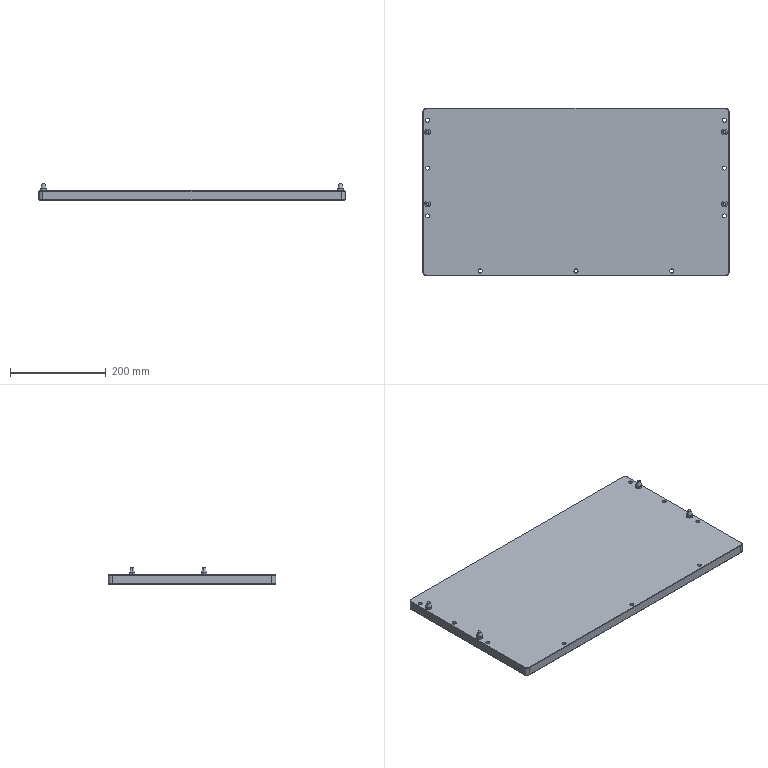Component | SolidWorks | AX00-102.1.1-1_AX00-101.1.1-1_04.1.1-1 | 5 solids | 76 faces | box 640 x 350 x 35 mm | volume 4471620 mm3 | cylinder 30 | plane 22 | cone 16 | torus 8 | commonest cylinder face diameters 8.5 x18 12 x8 16 x4
build123d program:
from build123d import *

# Parameters (mm, degrees)
SKETCH1_W             = 640
SKETCH1_H             = 350
BOSS_EXTRUDE1_DEPTH   = 10
FILLET1_R             = 8
CHAMFER1_SIZE         = 1
M10_TAPPED_HOLE1_D    = 8.5
SKETCH4_R             = 6
BOSS_EXTRUDE2_DEPTH   = 15
BOSS_EXTRUDE2_2_DEPTH = 15
BOSS_EXTRUDE2_3_DEPTH = 15
BOSS_EXTRUDE2_4_DEPTH = 15
CHAMFER2_SIZE         = 10
CHAMFER2_SIZE2        = 3
CHAMFER3_SIZE         = 10
CHAMFER3_SIZE2        = 3
CHAMFER4_SIZE         = 10
CHAMFER4_SIZE2        = 3
CHAMFER5_SIZE         = 10
CHAMFER5_SIZE2        = 3
FILLET2_R             = 5
FILLET3_R             = 5
FILLET4_R             = 5
FILLET5_R             = 5


with BuildPart() as part:
    # Sketch1 → Boss-Extrude1 (new, symmetric)
    with BuildSketch(Plane.XY):
        Rectangle(SKETCH1_W, SKETCH1_H)
    extrude(amount=BOSS_EXTRUDE1_DEPTH, both=True)

    # Fillet1
    fillet1_edges = [part.edges().sort_by_distance(p)[0] for p in [
        (320, -175, 0),
        (-320, -175, 0),
        (-320, 175, 0),
        (320, 175, 0),
    ]]
    fillet(fillet1_edges, radius=FILLET1_R)

    # Chamfer1
    chamfer1_edges = [part.edges().sort_by_distance(p)[0] for p in [
        (0, 175, -10),
        (0, 175, 10),
        (320, 0, -10),
        (0, -175, -10),
        (-320, 0, -10),
        (-317.657, -172.657, -10),
        (-317.657, 172.657, -10),
        (317.657, -172.657, -10),
        (317.657, 172.657, -10),
        (320, 0, 10),
        (-320, 0, 10),
        (0, -175, 10),
        (-317.657, -172.657, 10),
        (-317.657, 172.657, 10),
        (317.657, -172.657, 10),
        (317.657, 172.657, 10),
    ]]
    chamfer(chamfer1_edges, length=CHAMFER1_SIZE)

    # M10 Tapped Hole1 (through all)
    with Locations(Plane.XY.offset(10)):
        with Locations((310, 50), (310, -150), (-310, -150), (-310, 50), (310, -50), (-310, -50), (-200, 165), (0, 165), (200, 165)):
            Hole(M10_TAPPED_HOLE1_D / 2)


with BuildPart() as body_2:
    # Sketch4 → Boss-Extrude2 (new body)
    with BuildSketch(Plane.XY.offset(10)):
        with Locations((310, 25)):
            Circle(SKETCH4_R)
    extrude(amount=BOSS_EXTRUDE2_DEPTH)

    # Chamfer2
    chamfer2_edges = [body_2.edges().sort_by_distance(p)[0] for p in [
        (304, 25, 25),
    ]]
    chamfer2_side = [body_2.faces().sort_by_distance(p)[0] for p in [
        (304, 25, 17.5),
    ]]
    chamfer(chamfer2_edges, length=CHAMFER2_SIZE, length2=CHAMFER2_SIZE2, reference=chamfer2_side[0])

    # Fillet2
    fillet2_edges = [body_2.edges().sort_by_distance(p)[0] for p in [
        (304, 25, 15),
    ]]
    fillet(fillet2_edges, radius=FILLET2_R)


with BuildPart() as body_3:
    # Sketch4 → Boss-Extrude2 2 (new body)
    with BuildSketch(Plane.XY.offset(10)):
        with Locations((310, -125)):
            Circle(SKETCH4_R)
    extrude(amount=BOSS_EXTRUDE2_2_DEPTH)

    # Chamfer3
    chamfer3_edges = [body_3.edges().sort_by_distance(p)[0] for p in [
        (304, -125, 25),
    ]]
    chamfer3_side = [body_3.faces().sort_by_distance(p)[0] for p in [
        (304, -125, 17.5),
    ]]
    chamfer(chamfer3_edges, length=CHAMFER3_SIZE, length2=CHAMFER3_SIZE2, reference=chamfer3_side[0])

    # Fillet3
    fillet3_edges = [body_3.edges().sort_by_distance(p)[0] for p in [
        (304, -125, 15),
    ]]
    fillet(fillet3_edges, radius=FILLET3_R)


with BuildPart() as body_4:
    # Sketch4 → Boss-Extrude2 3 (new body)
    with BuildSketch(Plane.XY.offset(10)):
        with Locations((-310, 25)):
            Circle(SKETCH4_R)
    extrude(amount=BOSS_EXTRUDE2_3_DEPTH)

    # Chamfer4
    chamfer4_edges = [body_4.edges().sort_by_distance(p)[0] for p in [
        (-316, 25, 25),
    ]]
    chamfer4_side = [body_4.faces().sort_by_distance(p)[0] for p in [
        (-316, 25, 17.5),
    ]]
    chamfer(chamfer4_edges, length=CHAMFER4_SIZE, length2=CHAMFER4_SIZE2, reference=chamfer4_side[0])

    # Fillet4
    fillet4_edges = [body_4.edges().sort_by_distance(p)[0] for p in [
        (-316, 25, 15),
    ]]
    fillet(fillet4_edges, radius=FILLET4_R)


with BuildPart() as body_5:
    # Sketch4 → Boss-Extrude2 4 (new body)
    with BuildSketch(Plane.XY.offset(10)):
        with Locations((-310, -125)):
            Circle(SKETCH4_R)
    extrude(amount=BOSS_EXTRUDE2_4_DEPTH)

    # Chamfer5
    chamfer5_edges = [body_5.edges().sort_by_distance(p)[0] for p in [
        (-316, -125, 25),
    ]]
    chamfer5_side = [body_5.faces().sort_by_distance(p)[0] for p in [
        (-316, -125, 17.5),
    ]]
    chamfer(chamfer5_edges, length=CHAMFER5_SIZE, length2=CHAMFER5_SIZE2, reference=chamfer5_side[0])

    # Fillet5
    fillet5_edges = [body_5.edges().sort_by_distance(p)[0] for p in [
        (-316, -125, 15),
    ]]
    fillet(fillet5_edges, radius=FILLET5_R)


solid = Compound([part.part, body_2.part, body_3.part, body_4.part, body_5.part])

# Placed as in the assembly
solid = solid.moved(Location((228.631, 1338.364, 212.5), (0, 0, 180)))